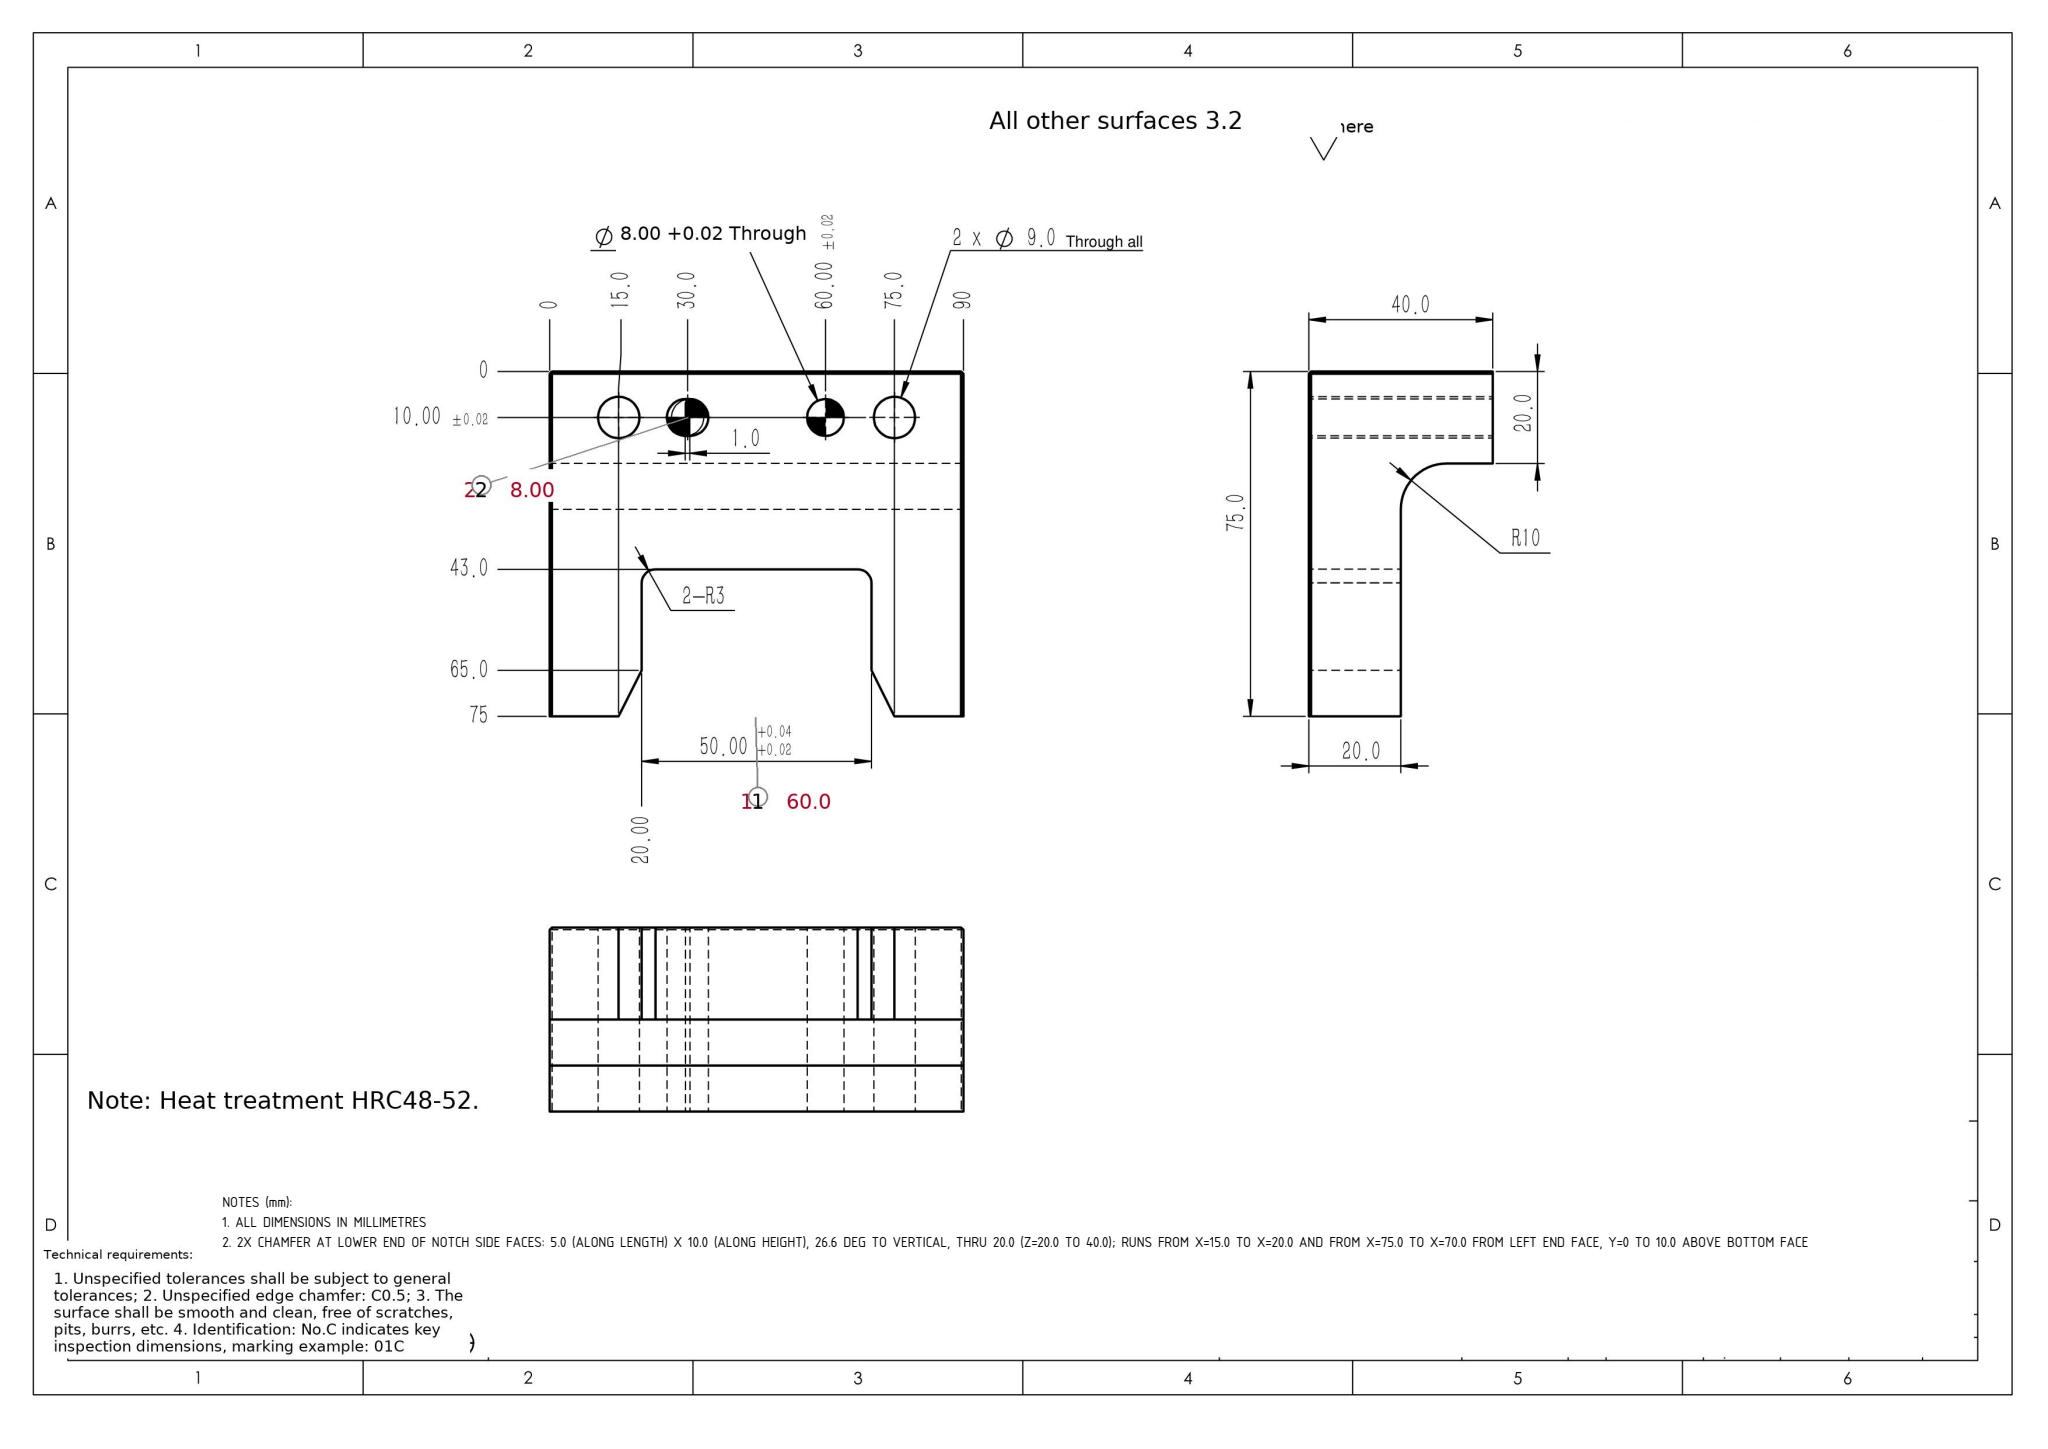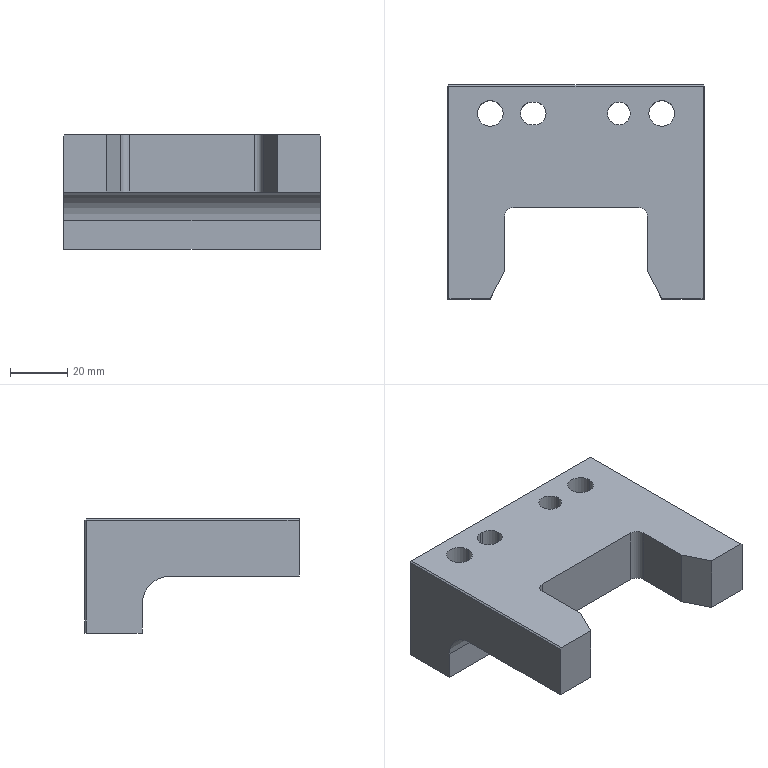Part | SolidWorks | mm | 1 solid | 35 faces | box 90 x 75 x 40 mm | volume 130538 mm3 | plane 23 | cylinder 12 | commonest cylinder face diameters 8 x5 9 x4 6 x2 20 x1
Drawing notes:
ALL DIMENSIONS IN MILLIMETRES | from the solid: STEP model units stated as mm
2X CHAMFER AT LOWER END OF NOTCH SIDE FACES: 5.0 (ALONG LENGTH) X 10.0 (ALONG HEIGHT), 26.6 DEG TO VERTICAL, THRU 20.0 (Z=20.0 TO 40.0); RUNS FROM X=15.0 TO X=20.0 AND FROM X=75.0 TO X=70.0 FROM LEFT END FACE, Y=0 TO 10.0 ABOVE BOTTOM FACE | from the solid: inclined_planes: angle_to_xyz_axes [26.6,63.4,90.0], bbox_from [15.0,0.0,20.0] and [70.0,0.0,20.0], size [5.0,10.0,20.0]
build123d program:
from build123d import *

# Parameters (mm, degrees)
SKETCH1_W            = 90
SKETCH1_H            = 75
BOSS_EXTRUDE1_DEPTH  = 10
SKETCH7_W            = 90
SKETCH7_H            = 20
BOSS_EXTRUDE2_DEPTH  = 20
M8_CLEARANCE_HOLE1_D = 9
SKETCH4_R            = 4
CUT_EXTRUDE1_DEPTH   = 71.931
SKETCH5_W            = 50
SKETCH5_H            = 32
CUT_EXTRUDE2_DEPTH   = 71.931
CUT_EXTRUDE3_DEPTH   = 71.931
FILLET1_R            = 3
FILLET2_R            = 10
CHAMFER1_SIZE        = 0.5


with BuildPart() as part:
    # Sketch1 → Boss-Extrude1 (new, symmetric)
    with BuildSketch(Plane.XY):
        Rectangle(SKETCH1_W, SKETCH1_H)
    extrude(amount=BOSS_EXTRUDE1_DEPTH, both=True)

    # Sketch7 → Boss-Extrude2 (add)
    with BuildSketch(Plane(origin=(0, 0, -10), x_dir=(-1, 0, 0), z_dir=(0, 0, -1))):
        with Locations((0, 27.5)):
            Rectangle(SKETCH7_W, SKETCH7_H)
    extrude(amount=BOSS_EXTRUDE2_DEPTH)

    # M8 Clearance Hole1 (through all)
    with Locations(Plane.XY.offset(10)):
        with Locations((30, 27.5), (-30, 27.5)):
            Hole(M8_CLEARANCE_HOLE1_D / 2)

    # Sketch4 → Cut-Extrude1 (cut, through all)
    with BuildSketch(Plane.XY.offset(10)):
        with Locations((15, 27.5)):
            Circle(SKETCH4_R)
        with BuildLine():
            Line((-14.5, 23.5), (-15.5, 23.5))
            ThreePointArc((-15.5, 23.5), (-19.5, 27.5), (-15.5, 31.5))
            Line((-15.5, 31.5), (-14.5, 31.5))
            ThreePointArc((-14.5, 31.5), (-10.5, 27.5), (-14.5, 23.5))
        make_face()
    extrude(amount=-CUT_EXTRUDE1_DEPTH, mode=Mode.SUBTRACT)

    # Sketch5 → Cut-Extrude2 (cut, through all)
    with BuildSketch(Plane.XY.offset(10)):
        with Locations((0, -21.5)):
            Rectangle(SKETCH5_W, SKETCH5_H)
    extrude(amount=-CUT_EXTRUDE2_DEPTH, mode=Mode.SUBTRACT)

    # Sketch6 → Cut-Extrude3 (cut, through all)
    with BuildSketch(Plane.XY.offset(10)):
        Polygon((25, -37.5), (25, -27.5), (30, -37.5), align=None)
        Polygon((-30, -37.5), (-25, -37.5), (-25, -27.5), align=None)
    extrude(amount=-CUT_EXTRUDE3_DEPTH, mode=Mode.SUBTRACT)

    # Fillet1
    fillet1_edges = [part.edges().sort_by_distance(p)[0] for p in [
        (-25, -5.5, 0),
        (25, -5.5, 0),
    ]]
    fillet(fillet1_edges, radius=FILLET1_R)

    # Fillet2
    fillet2_edges = [part.edges().sort_by_distance(p)[0] for p in [
        (0, 17.5, -10),
    ]]
    fillet(fillet2_edges, radius=FILLET2_R)

    # Chamfer1
    chamfer1_edges = [part.edges().sort_by_distance(p)[0] for p in [
        (-45, 0, 10),
        (45, 0, 10),
        (0, 37.5, 10),
        (-45, 37.5, -10),
        (45, 37.5, -10),
    ]]
    chamfer(chamfer1_edges, length=CHAMFER1_SIZE)


solid = part.part